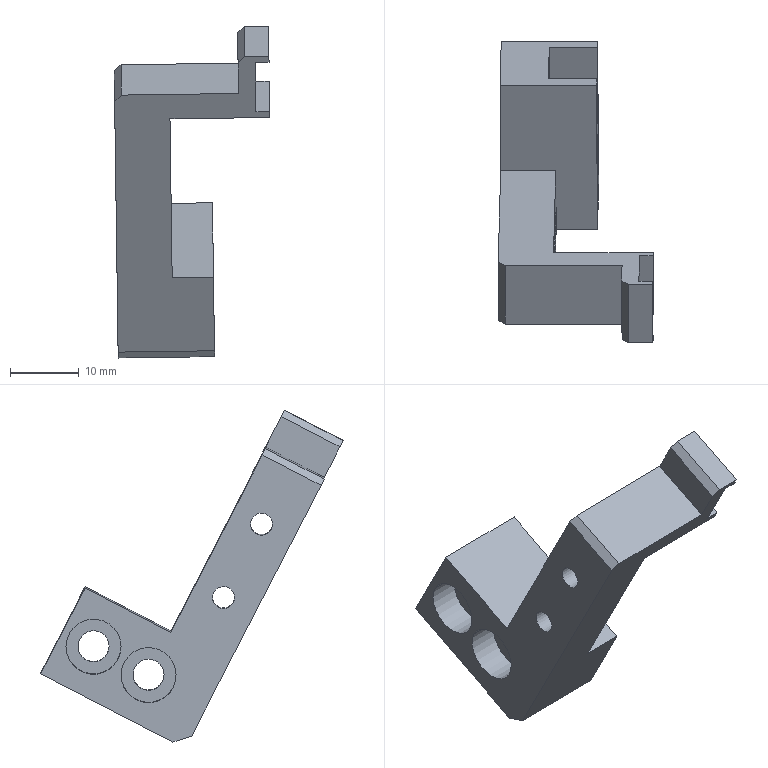Component | SolidWorks | 2018SOLIDWORKS1400000012-1 | 1 solid | 43 faces | box 22.6 x 43.92 x 48.22 mm | volume 5344 mm3 | plane 27 | cylinder 16 | commonest cylinder face diameters 3.2 x4 8 x4 4.5 x4 6 x2 2.5 x2 | material 45 Steel
build123d program:
from build123d import *

# Parameters (mm, degrees)
SKETCH1_W                                       = 23.6
SKETCH1_H                                       = 14
BOSS_EXTRUDE1_DEPTH                             = 14
M4_HEX_SOCKET_HEAD_CAP_SCREW_CBORE1_D           = 4.5
M4_HEX_SOCKET_HEAD_CAP_SCREW_CBORE1_CBORE_D     = 8
M4_HEX_SOCKET_HEAD_CAP_SCREW_CBORE1_CBORE_DEPTH = 4.4
CUT_EXTRUDE18_DEPTH                             = 7
SKETCH36_W                                      = 9.6
SKETCH36_H                                      = 8
BOSS_EXTRUDE2_DEPTH                             = 36
SKETCH37_W                                      = 9.6
SKETCH37_H                                      = 10
BOSS_EXTRUDE3_DEPTH                             = 14.5
SKETCH38_W                                      = 9.6
SKETCH38_H                                      = 8
CUT_EXTRUDE19_DEPTH                             = 2
CHAMFER1_SIZE                                   = 2
SKETCH39_R                                      = 1.6
CUT_EXTRUDE20_DEPTH                             = 15
SKETCH40_R                                      = 3
CUT_EXTRUDE21_DEPTH                             = 6
SKETCH41_W                                      = 18
SKETCH41_H                                      = 23.935
CUT_EXTRUDE22_DEPTH                             = 15
CHAMFER2_SIZE                                   = 1
CHAMFER3_SIZE                                   = 2


with BuildPart() as part:
    # Sketch1 → Boss-Extrude1 (new body)
    with BuildSketch(Plane.XY):
        Rectangle(SKETCH1_W, SKETCH1_H)
    extrude(amount=BOSS_EXTRUDE1_DEPTH)

    # M4 Hex Socket Head Cap Screw CBORE1 (through all)
    with Locations(Plane.XY.offset(14)):
        with Locations((-6.8, 0), (2.2, 0)):
            CounterBoreHole(M4_HEX_SOCKET_HEAD_CAP_SCREW_CBORE1_D / 2, M4_HEX_SOCKET_HEAD_CAP_SCREW_CBORE1_CBORE_D / 2, M4_HEX_SOCKET_HEAD_CAP_SCREW_CBORE1_CBORE_DEPTH)

    # Sketch35 → Cut-Extrude18 (cut)
    with BuildSketch(Plane(origin=(0, 0, 0), x_dir=(-1, 0, 0), z_dir=(0, 0, -1))):
        with BuildLine():
            Line((11.8, 5), (-6.25, 5))
            ThreePointArc((-6.25, 5), (-8.484, 5.771), (-7.2, 3.787))
            Line((-7.2, 3.787), (-7.2, -3.787))
            ThreePointArc((-7.2, -3.787), (-8.484, -5.771), (-6.25, -5))
            Line((-6.25, -5), (11.8, -5))
            Line((11.8, -5), (11.8, 5))
        make_face()
    extrude(amount=-CUT_EXTRUDE18_DEPTH, mode=Mode.SUBTRACT)

    # Sketch36 → Boss-Extrude2 (add)
    with BuildSketch(Plane(origin=(0, 7, 0), x_dir=(1, 0, 0), z_dir=(0, 1, 0))):
        with Locations((7, -10)):
            Rectangle(SKETCH36_W, SKETCH36_H)
    extrude(amount=BOSS_EXTRUDE2_DEPTH)

    # Sketch37 → Boss-Extrude3 (add)
    with BuildSketch(Plane(origin=(0, 0, 6), x_dir=(-1, 0, 0), z_dir=(0, 0, -1))):
        with Locations((-7, 38)):
            Rectangle(SKETCH37_W, SKETCH37_H)
    extrude(amount=BOSS_EXTRUDE3_DEPTH)

    # Sketch38 → Cut-Extrude19 (cut)
    with BuildSketch(Plane(origin=(0, 0, -8.5), x_dir=(-1, 0, 0), z_dir=(0, 0, -1))):
        with Locations((-7, 38)):
            Rectangle(SKETCH38_W, SKETCH38_H)
    extrude(amount=-CUT_EXTRUDE19_DEPTH, mode=Mode.SUBTRACT)

    # Chamfer1
    chamfer1_edges = [part.edges().sort_by_distance(p)[0] for p in [
        (7, 43, 14),
    ]]
    chamfer(chamfer1_edges, length=CHAMFER1_SIZE)

    # Sketch39 → Cut-Extrude20 (cut)
    with BuildSketch(Plane(origin=(0, 0, 6), x_dir=(-1, 0, 0), z_dir=(0, 0, -1))):
        with Locations((-6.7, 27)):
            Circle(SKETCH39_R)
        with Locations((-6.7, 15)):
            Circle(SKETCH39_R)
    extrude(amount=-CUT_EXTRUDE20_DEPTH, mode=Mode.SUBTRACT)

    # Sketch40 → Cut-Extrude21 (cut)
    with BuildSketch(Plane(origin=(0, 0, 6), x_dir=(-1, 0, 0), z_dir=(0, 0, -1))):
        with Locations((-6.7, 21)):
            Circle(SKETCH40_R)
    extrude(amount=-CUT_EXTRUDE21_DEPTH, mode=Mode.SUBTRACT)

    # Sketch41 → Cut-Extrude22 (cut)
    with BuildSketch(Plane(origin=(11.8, 0, 0), x_dir=(0, 0, -1), z_dir=(1, 0, 0))):
        with Locations((-5, 48.967)):
            Rectangle(SKETCH41_W, SKETCH41_H)
    extrude(amount=-CUT_EXTRUDE22_DEPTH, mode=Mode.SUBTRACT)

    # Chamfer2
    chamfer2_edges = [part.edges().sort_by_distance(p)[0] for p in [
        (7, 43, -4),
        (7, 37, 14),
    ]]
    chamfer(chamfer2_edges, length=CHAMFER2_SIZE)

    # Chamfer3
    chamfer3_edges = [part.edges().sort_by_distance(p)[0] for p in [
        (11.8, -7, 7),
    ]]
    chamfer(chamfer3_edges, length=CHAMFER3_SIZE)


solid = part.part

# Placed as in the assembly
solid = solid.moved(Location((82.775, -82.786, 161.423), (-180, -89.207, 62.677)))